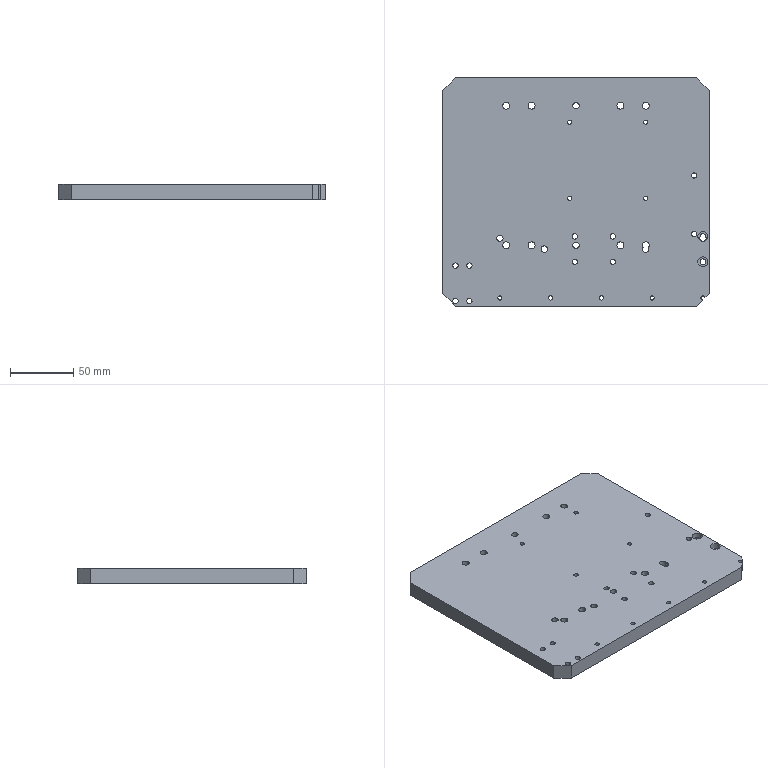Component | SolidWorks | 01-1111-1 | 1 solid | 117 faces | box 210 x 180 x 12 mm | volume 442192 mm3 | cylinder 96 | plane 21 | commonest cylinder face diameters 4.2 x20 3.3 x18 10 x18 5.5 x17 5 x14 4.5 x5 8 x4 | material 1060 Alloy
build123d program:
from build123d import *

# Parameters (mm, degrees)
SKETCH2_W                                       = 210
SKETCH2_H                                       = 180
BOSS_EXTRUDE1_DEPTH                             = 6
M5_HEX_SOCKET_HEAD_CAP_SCREW_CBORE2_D           = 5.5
M5_HEX_SOCKET_HEAD_CAP_SCREW_CBORE2_CBORE_D     = 10
M5_HEX_SOCKET_HEAD_CAP_SCREW_CBORE2_CBORE_DEPTH = 5.4
SIZE_MM_DOWEL_HOLE2_D                           = 5
CHAMFER1_SIZE                                   = 10
M5_TAPPED_HOLE1_D                               = 4.2
M4_TAPPED_HOLE1_D                               = 3.3
M5_TAPPED_HOLE3_D                               = 4.2
SIZE_MM_DOWEL_HOLE3_D                           = 5
M5_TAPPED_HOLE2_D                               = 4.2
M4_HEX_SOCKET_HEAD_CAP_SCREW_CBORE1_D           = 4.5
M4_HEX_SOCKET_HEAD_CAP_SCREW_CBORE1_CBORE_D     = 8
M4_HEX_SOCKET_HEAD_CAP_SCREW_CBORE1_CBORE_DEPTH = 4.4
M4_TAPPED_HOLE2_D                               = 3.3


with BuildPart() as part:
    # Sketch2 → Boss-Extrude1 (new, symmetric)
    with BuildSketch(Plane.XY):
        Rectangle(SKETCH2_W, SKETCH2_H)
    extrude(amount=BOSS_EXTRUDE1_DEPTH, both=True)

    # M5 Hex Socket Head Cap Screw CBORE2 (through all)
    with Locations(Plane(origin=(0, 0, -6), x_dir=(-1, 0, 0), z_dir=(0, 0, -1))):
        with Locations((55, 68), (35, 68), (-35, 68), (-55, 68), (-55, -42), (-35, -42), (35, -42), (55, -42)):
            CounterBoreHole(M5_HEX_SOCKET_HEAD_CAP_SCREW_CBORE2_D / 2, M5_HEX_SOCKET_HEAD_CAP_SCREW_CBORE2_CBORE_D / 2, M5_HEX_SOCKET_HEAD_CAP_SCREW_CBORE2_CBORE_DEPTH)

    # Size mm Dowel Hole2 (through all)
    with Locations(Plane(origin=(0, 0, -6), x_dir=(-1, 0, 0), z_dir=(0, 0, -1))):
        with Locations((0, 68), (0, -42)):
            Hole(SIZE_MM_DOWEL_HOLE2_D / 2)

    # Chamfer1
    chamfer1_edges = [part.edges().sort_by_distance(p)[0] for p in [
        (105, -90, 0),
        (-105, -90, 0),
        (-105, 90, 0),
        (105, 90, 0),
    ]]
    chamfer(chamfer1_edges, length=CHAMFER1_SIZE)

    # M5 Tapped Hole1 (through all)
    with Locations(Plane(origin=(0, 0, -6), x_dir=(-1, 0, 0), z_dir=(0, 0, -1))):
        with Locations((-29, -35), (-29, -55), (1, -55), (1, -35)):
            Hole(M5_TAPPED_HOLE1_D / 2)

    # M4 Tapped Hole1 (through all)
    with Locations(Plane(origin=(0, 0, -6), x_dir=(-1, 0, 0), z_dir=(0, 0, -1))):
        with Locations((60, -83.5), (60, -106.5), (20, -83.5), (20, -106.5), (-20, -83.5), (-20, -106.5), (-60, -83.5), (-60, -106.5), (-100, -106.5), (-100, -83.5)):
            Hole(M4_TAPPED_HOLE1_D / 2)

    # M5 Tapped Hole3 (through all)
    with Locations(Plane.XY.offset(6)):
        with Locations((-84, -86), (-95, -86), (-95, -58), (-84, -58)):
            Hole(M5_TAPPED_HOLE3_D / 2)

    # Size mm Dowel Hole3 (through all)
    with Locations(Plane(origin=(0, 0, -6), x_dir=(-1, 0, 0), z_dir=(0, 0, -1))):
        with Locations((-55, -45), (25, -45), (-100, -36.5), (60, -36.5)):
            Hole(SIZE_MM_DOWEL_HOLE3_D / 2)

    # M5 Tapped Hole2 (through all)
    with Locations(Plane(origin=(0, 0, -6), x_dir=(-1, 0, 0), z_dir=(0, 0, -1))):
        with Locations((-93, 13), (-93, -33)):
            Hole(M5_TAPPED_HOLE2_D / 2)

    # M4 Hex Socket Head Cap Screw CBORE1 (through all)
    with Locations(Plane.XY.offset(6)):
        with Locations((100, -55), (100, -35)):
            CounterBoreHole(M4_HEX_SOCKET_HEAD_CAP_SCREW_CBORE1_D / 2, M4_HEX_SOCKET_HEAD_CAP_SCREW_CBORE1_CBORE_D / 2, M4_HEX_SOCKET_HEAD_CAP_SCREW_CBORE1_CBORE_DEPTH)

    # M4 Tapped Hole2 (through all)
    with Locations(Plane(origin=(0, 0, -6), x_dir=(-1, 0, 0), z_dir=(0, 0, -1))):
        with Locations((5, 55), (-55, 55), (-55, -5), (5, -5)):
            Hole(M4_TAPPED_HOLE2_D / 2)


solid = part.part